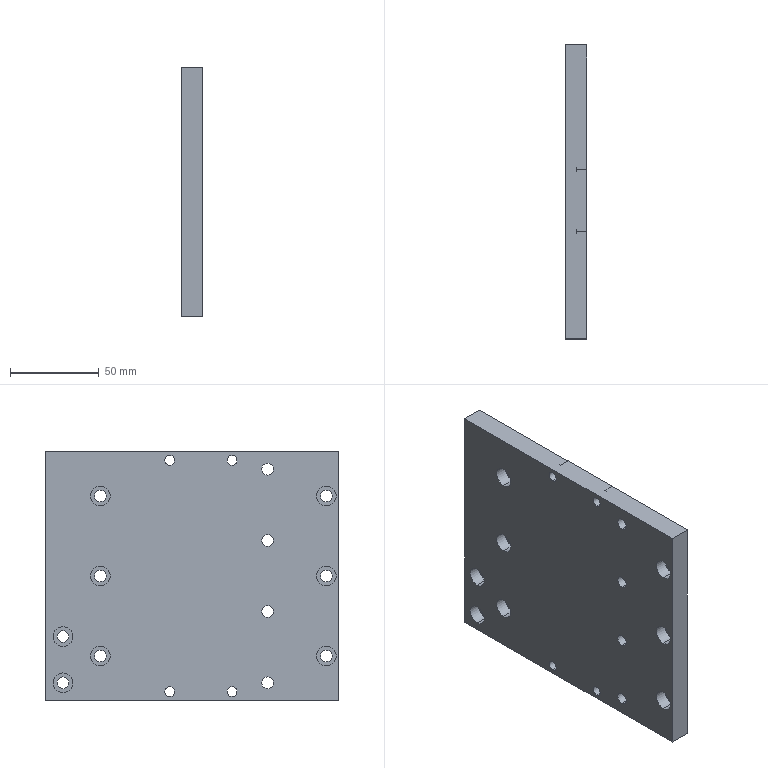Component | SolidWorks | SL021-102-4066.SL4PRT-1 | 1 solid | 86 faces | box 12 x 165 x 140 mm | volume 265096 mm3 | cylinder 64 | plane 22 | commonest cylinder face diameters 11 x24 6.6 x24 9.5 x8 5.5 x8 | material AL6061
build123d program:
from build123d import *

# Parameters (mm, degrees)
SKETCH1_W                                          = 140
SKETCH1_H                                          = 165
BOSS_EXTRUDE1_DEPTH                                = 6
HOLE_SIZE_ACCORDING_TO_TYPE_1_OF_HEXAG_D           = 6.6
HOLE_SIZE_ACCORDING_TO_TYPE_1_OF_HEXAG_CBORE_D     = 11
HOLE_SIZE_ACCORDING_TO_TYPE_1_OF_HEXAG_CBORE_DEPTH = 6.8
HOLE_SIZE_ACCORDING_TO_TYPE_2_OF_HEXAG_D           = 5.5
HOLE_SIZE_ACCORDING_TO_TYPE_2_OF_HEXAG_CBORE_D     = 9.5
HOLE_SIZE_ACCORDING_TO_TYPE_2_OF_HEXAG_CBORE_DEPTH = 5.7
HOLE_SIZE_ACCORDING_TO_TYPE_3_OF_HEXAG_D           = 6.6
HOLE_SIZE_ACCORDING_TO_TYPE_3_OF_HEXAG_CBORE_D     = 11
HOLE_SIZE_ACCORDING_TO_TYPE_3_OF_HEXAG_CBORE_DEPTH = 6.8
HOLE_SIZE_ACCORDING_TO_TYPE_4_OF_HEXAG_D           = 6.6
HOLE_SIZE_ACCORDING_TO_TYPE_4_OF_HEXAG_CBORE_D     = 11
HOLE_SIZE_ACCORDING_TO_TYPE_4_OF_HEXAG_CBORE_DEPTH = 6.8


with BuildPart() as part:
    # Sketch1 → Boss-Extrude1 (new, symmetric)
    with BuildSketch(Plane.XY):
        Rectangle(SKETCH1_W, SKETCH1_H)
    extrude(amount=BOSS_EXTRUDE1_DEPTH, both=True)

    # Hole Size _According to_ Type 1 of Hexag (through all)
    with Locations(Plane(origin=(0, 0, -6), x_dir=(-1, 0, 0), z_dir=(0, 0, -1))):
        with Locations((-45, 51.5), (0, 51.5), (45, 51.5), (-45, -75.5), (0, -75.5), (45, -75.5)):
            CounterBoreHole(HOLE_SIZE_ACCORDING_TO_TYPE_1_OF_HEXAG_D / 2, HOLE_SIZE_ACCORDING_TO_TYPE_1_OF_HEXAG_CBORE_D / 2, HOLE_SIZE_ACCORDING_TO_TYPE_1_OF_HEXAG_CBORE_DEPTH)

    # Hole Size _According to_ Type 2 of Hexag (through all)
    with Locations(Plane.XY.offset(6)):
        with Locations((-65, 12.5), (-65, -22.5), (65, 12.5), (65, -22.5)):
            CounterBoreHole(HOLE_SIZE_ACCORDING_TO_TYPE_2_OF_HEXAG_D / 2, HOLE_SIZE_ACCORDING_TO_TYPE_2_OF_HEXAG_CBORE_D / 2, HOLE_SIZE_ACCORDING_TO_TYPE_2_OF_HEXAG_CBORE_DEPTH)

    # Hole Size _According to_ Type 3 of Hexag (through all)
    with Locations(Plane(origin=(0, 0, -6), x_dir=(-1, 0, 0), z_dir=(0, 0, -1))):
        with Locations((-60, 72.5), (-34, 72.5)):
            CounterBoreHole(HOLE_SIZE_ACCORDING_TO_TYPE_3_OF_HEXAG_D / 2, HOLE_SIZE_ACCORDING_TO_TYPE_3_OF_HEXAG_CBORE_D / 2, HOLE_SIZE_ACCORDING_TO_TYPE_3_OF_HEXAG_CBORE_DEPTH)

    # Hole Size _According to_ Type 4 of Hexag (through all)
    with Locations(Plane.XY.offset(6)):
        with Locations((-60, -42.5), (-20, -42.5), (20, -42.5), (60, -42.5)):
            CounterBoreHole(HOLE_SIZE_ACCORDING_TO_TYPE_4_OF_HEXAG_D / 2, HOLE_SIZE_ACCORDING_TO_TYPE_4_OF_HEXAG_CBORE_D / 2, HOLE_SIZE_ACCORDING_TO_TYPE_4_OF_HEXAG_CBORE_DEPTH)


solid = part.part

# Placed as in the assembly
solid = solid.moved(Location((19.837, 27.001, -151.378), (0, 90, 0)))